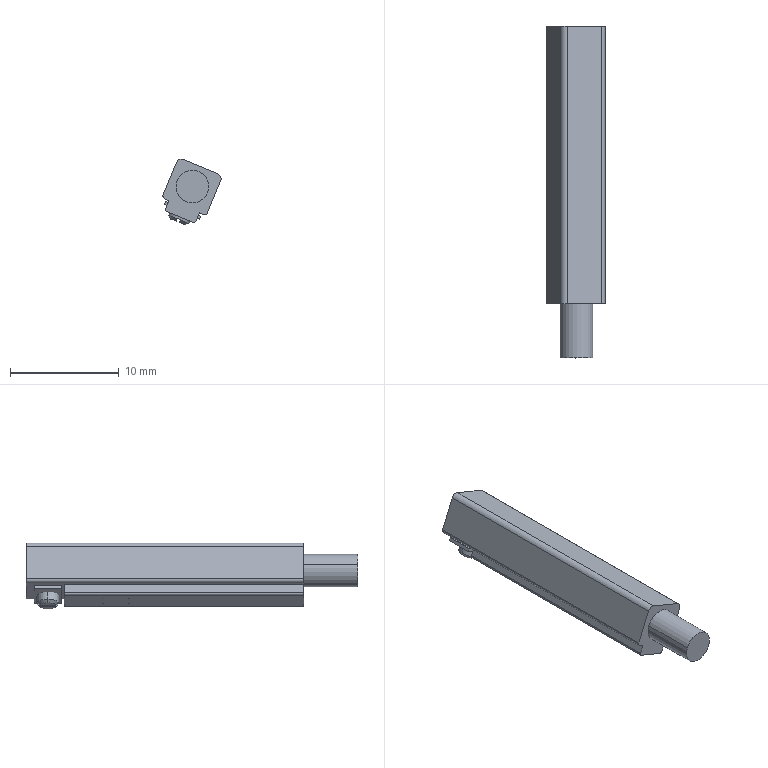Component | SolidWorks | ACQS_63x50_G_2_50-1_CS1_G-2 | 1 solid | 46 faces | box 5.35 x 30.5 x 6.06 mm | volume 552 mm3 | plane 27 | cylinder 16 | cone 3 | commonest cylinder face diameters 2 x4 0.5 x4 3 x2 1 x2 0.6 x2 0.4 x2
build123d program:
from build123d import *

# Parameters (mm, degrees)
BOSS_EXTRUDE1_DEPTH      = 25.5
SKETCH2_W                = 3
SKETCH2_H                = 1
CUT_EXTRUDE1_DEPTH       = 3.5
CUT_EXTRUDE2_DEPTH       = 1.25
CUT_EXTRUDE2_DEPTH_BACK  = 1.25
SKETCH4_W                = 0.3
SKETCH4_H                = 0.3
BOSS_EXTRUDE2_DEPTH      = 1.25
BOSS_EXTRUDE2_DEPTH_BACK = 1.25
SKETCH5_W                = 4.4
SKETCH5_H                = 0.3
SKETCH6_R                = 1.5
BOSS_EXTRUDE3_DEPTH      = 30.5
CUT_EXTRUDE3_DEPTH       = 0.01
SLOTLIPRELIEF_BY         = 0.45
SLOTLIPRELIEF_2_BY       = 0.45


with BuildPart() as part:
    # Sketch1 → Boss-Extrude1 (new body)
    with BuildSketch(Plane(origin=(0, 0, 0), x_dir=(0, 0, -1), z_dir=(1, 0, 0))):
        with BuildLine():
            Line((-1.7, 0), (1.7, 0))
            ThreePointArc((1.7, 0), (2.054, 0.1464), (2.2, 0.5))
            Line((2.2, 0.5), (2.2, 3.7))
            ThreePointArc((2.2, 3.7), (2.112, 3.912), (1.9, 4))
            Line((1.9, 4), (1.5, 4))
            Line((1.5, 4), (1.5, 4.8))
            ThreePointArc((1.5, 4.8), (1.441, 4.941), (1.3, 5))
            Line((1.3, 5), (-1.3, 5))
            ThreePointArc((-1.3, 5), (-1.441, 4.941), (-1.5, 4.8))
            Line((-1.5, 4.8), (-1.5, 4))
            Line((-1.5, 4), (-1.9, 4))
            ThreePointArc((-1.9, 4), (-2.112, 3.912), (-2.2, 3.7))
            Line((-2.2, 3.7), (-2.2, 0.5))
            ThreePointArc((-2.2, 0.5), (-2.054, 0.1464), (-1.7, 0))
        make_face()
    extrude(amount=BOSS_EXTRUDE1_DEPTH)

    # Sketch2 → Cut-Extrude1 (cut)
    with BuildSketch(Plane(origin=(0, 0, 0), x_dir=(0, 0, -1), z_dir=(1, 0, 0))):
        with Locations((0, 4.5)):
            Rectangle(SKETCH2_W, SKETCH2_H)
    extrude(amount=CUT_EXTRUDE1_DEPTH, mode=Mode.SUBTRACT)

    # Sketch3 → Revolve1 (revolve)
    with BuildSketch(Plane(origin=(2, 0, 0), x_dir=(0, 0, -1), z_dir=(1, 0, 0)), mode=Mode.PRIVATE) as revolve1_sk:
        Polygon((0, 5.5), (0.7545, 5.5), (1, 5.255), (1, 3.9), (0, 3.9), align=None)
    revolve(revolve1_sk.sketch.rotate(Axis((2, 3.9, 0), (0, 1, 0)), 180), axis=Axis((2, 3.9, 0), (0, 1, 0)))

    # Sketch4 → Cut-Extrude2 (cut, two sides: drawn at the far end of the back side and taken through both)
    with BuildSketch(Plane(origin=(2, 0, 0), x_dir=(0, 0, -1), z_dir=(1, 0, 0)).offset(-CUT_EXTRUDE2_DEPTH_BACK)):
        with Locations((0, 5.35)):
            Rectangle(SKETCH4_W, SKETCH4_H)
    extrude(amount=CUT_EXTRUDE2_DEPTH + CUT_EXTRUDE2_DEPTH_BACK, mode=Mode.SUBTRACT)

    # Sketch5 → Boss-Extrude2 (add, two sides: drawn at the far end of the back side and taken through both)
    with BuildSketch(Plane(origin=(2, 0, 0), x_dir=(0, 0, -1), z_dir=(1, 0, 0)).offset(-BOSS_EXTRUDE2_DEPTH_BACK)):
        with Locations((0, 4.35)):
            Rectangle(SKETCH5_W, SKETCH5_H)
    extrude(amount=BOSS_EXTRUDE2_DEPTH + BOSS_EXTRUDE2_DEPTH_BACK)

    # Sketch6 → Boss-Extrude3 (add)
    with BuildSketch(Plane(origin=(0, 0, 0), x_dir=(0, 0, -1), z_dir=(1, 0, 0))):
        with Locations(Location((0, 2, 0), (0, 0, 180))):
            Circle(SKETCH6_R)
    extrude(amount=BOSS_EXTRUDE3_DEPTH)

    # Sketch7 → Cut-Extrude3 (cut)
    with BuildSketch(Plane(origin=(0, 5, 0), x_dir=(-1, 0, 0), z_dir=(0, 1, 0))):
        with BuildLine():
            Line((-7.25, 0.75), (-9.25, 0.75))
            ThreePointArc((-9.25, 0.75), (-9.427, 0.6768), (-9.5, 0.5))
            Line((-9.5, 0.5), (-9.5, -0.5))
            ThreePointArc((-9.5, -0.5), (-9.427, -0.6768), (-9.25, -0.75))
            Line((-9.25, -0.75), (-7.25, -0.75))
            ThreePointArc((-7.25, -0.75), (-7.073, -0.6768), (-7, -0.5))
            Line((-7, -0.5), (-7, 0.5))
            ThreePointArc((-7, 0.5), (-7.073, 0.6768), (-7.25, 0.75))
        make_face()
    extrude(amount=-CUT_EXTRUDE3_DEPTH, mode=Mode.SUBTRACT)

    # SlotLipRelief: a face moved inward by 0.45
    extrude(part.faces().sort_by_distance((2, 4.35, 2.2))[0], amount=SLOTLIPRELIEF_BY, dir=(0, 0, -1), mode=Mode.SUBTRACT)

    # SlotLipRelief 2: a face moved inward by 0.45
    extrude(part.faces().sort_by_distance((2, 4.35, -2.2))[0], amount=SLOTLIPRELIEF_2_BY, dir=(0, 0, 1), mode=Mode.SUBTRACT)


solid = part.part

# Placed as in the assembly
solid = solid.moved(Location((-580.197, -155.873, 2365.602), (-180, 67.5, 90)))